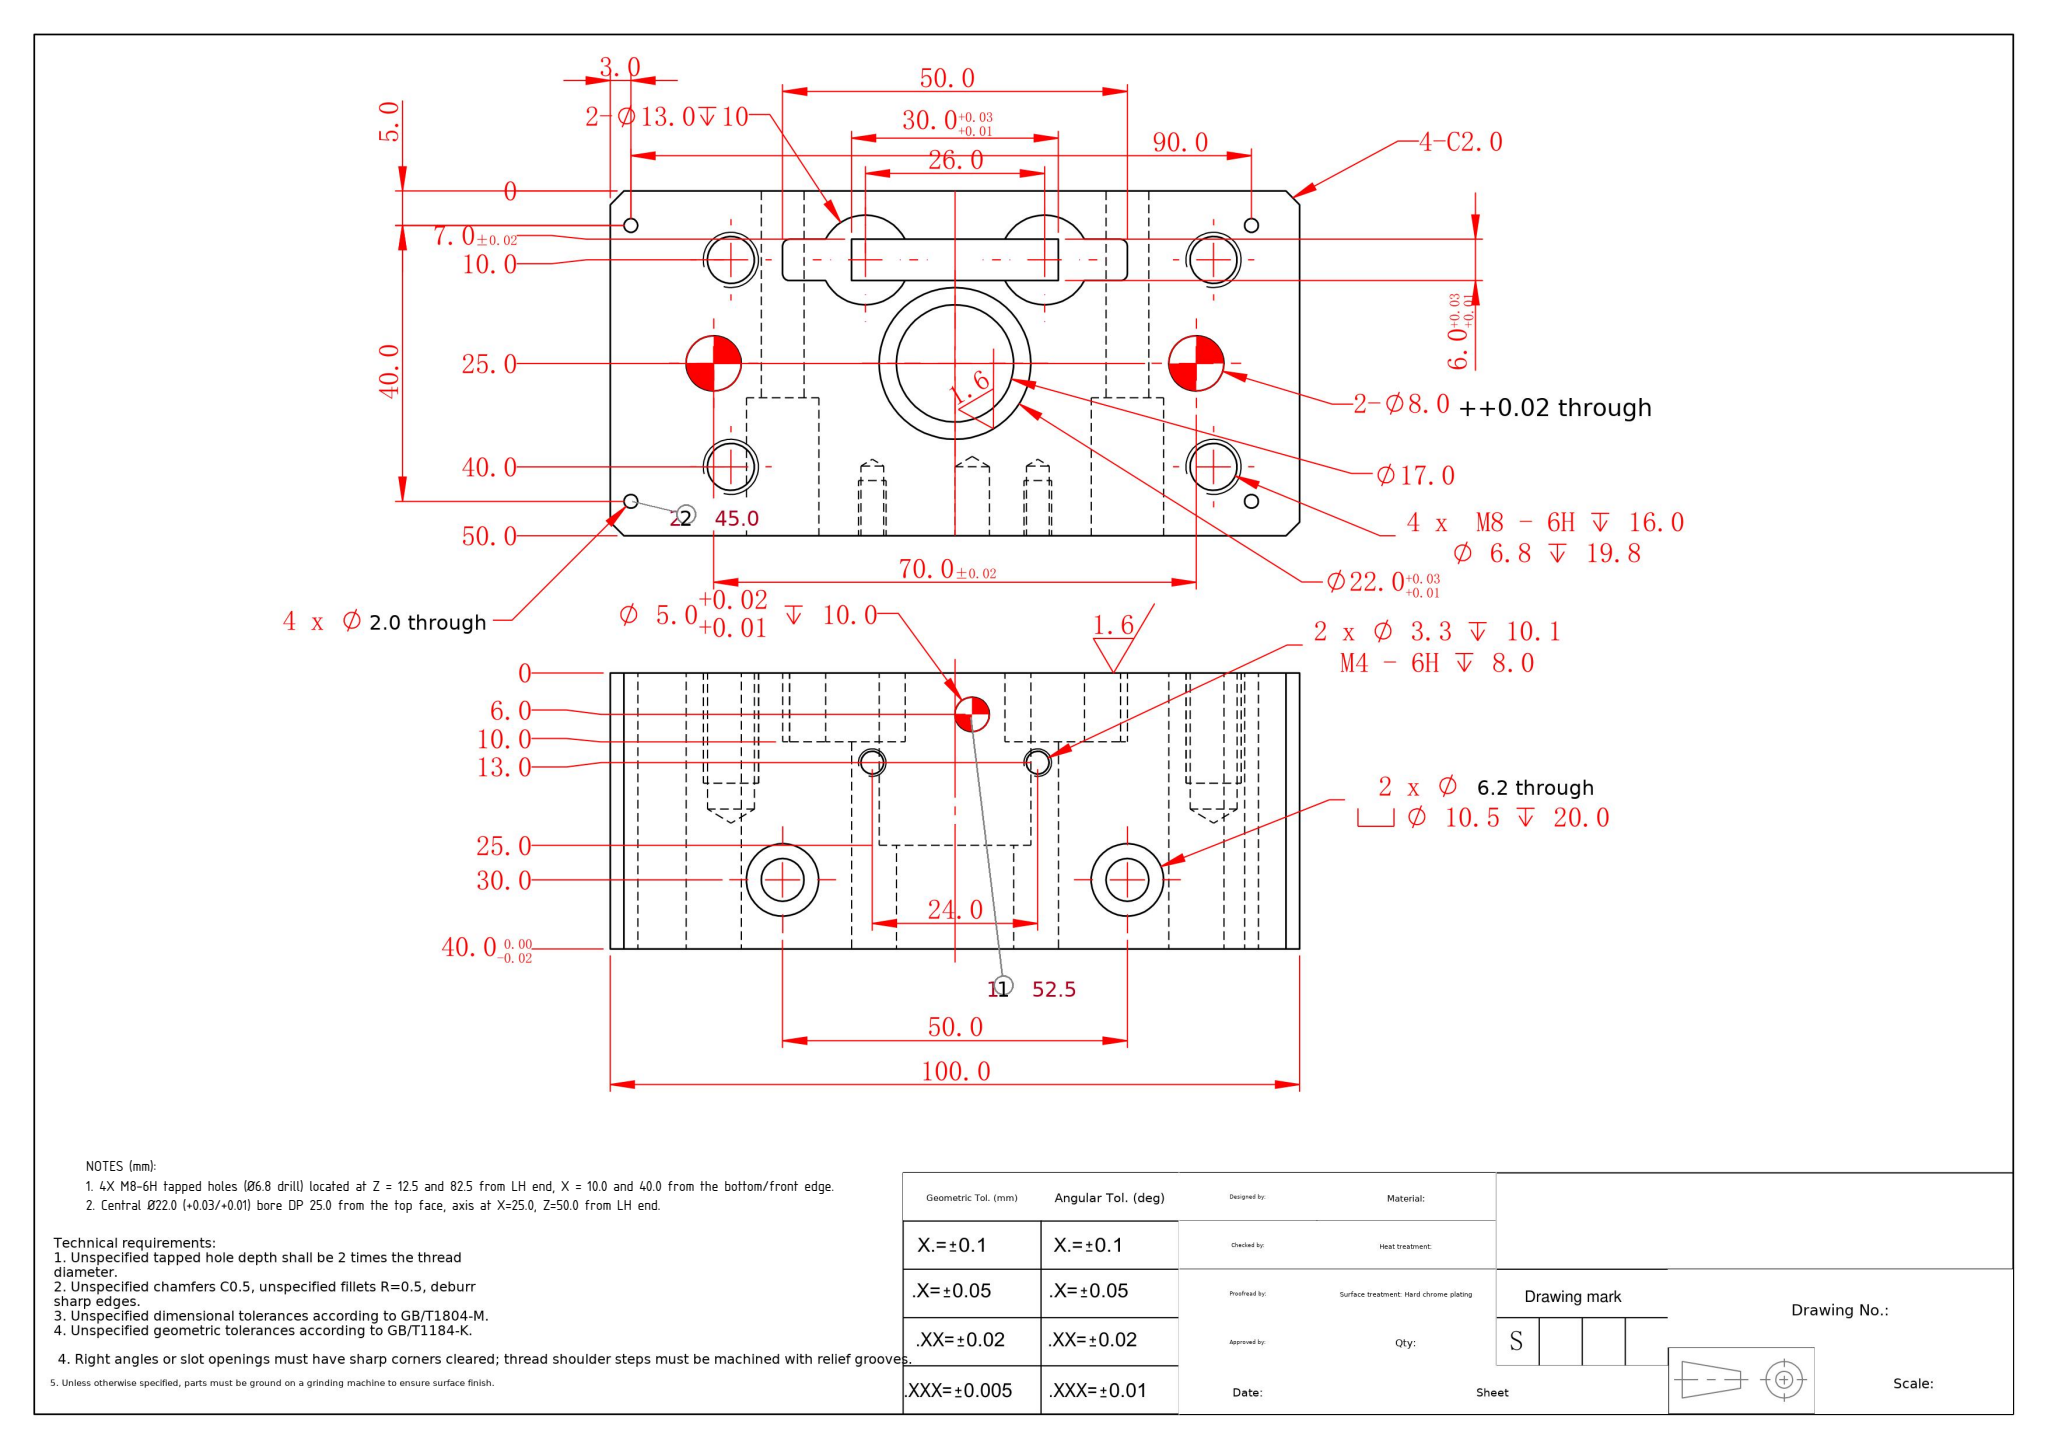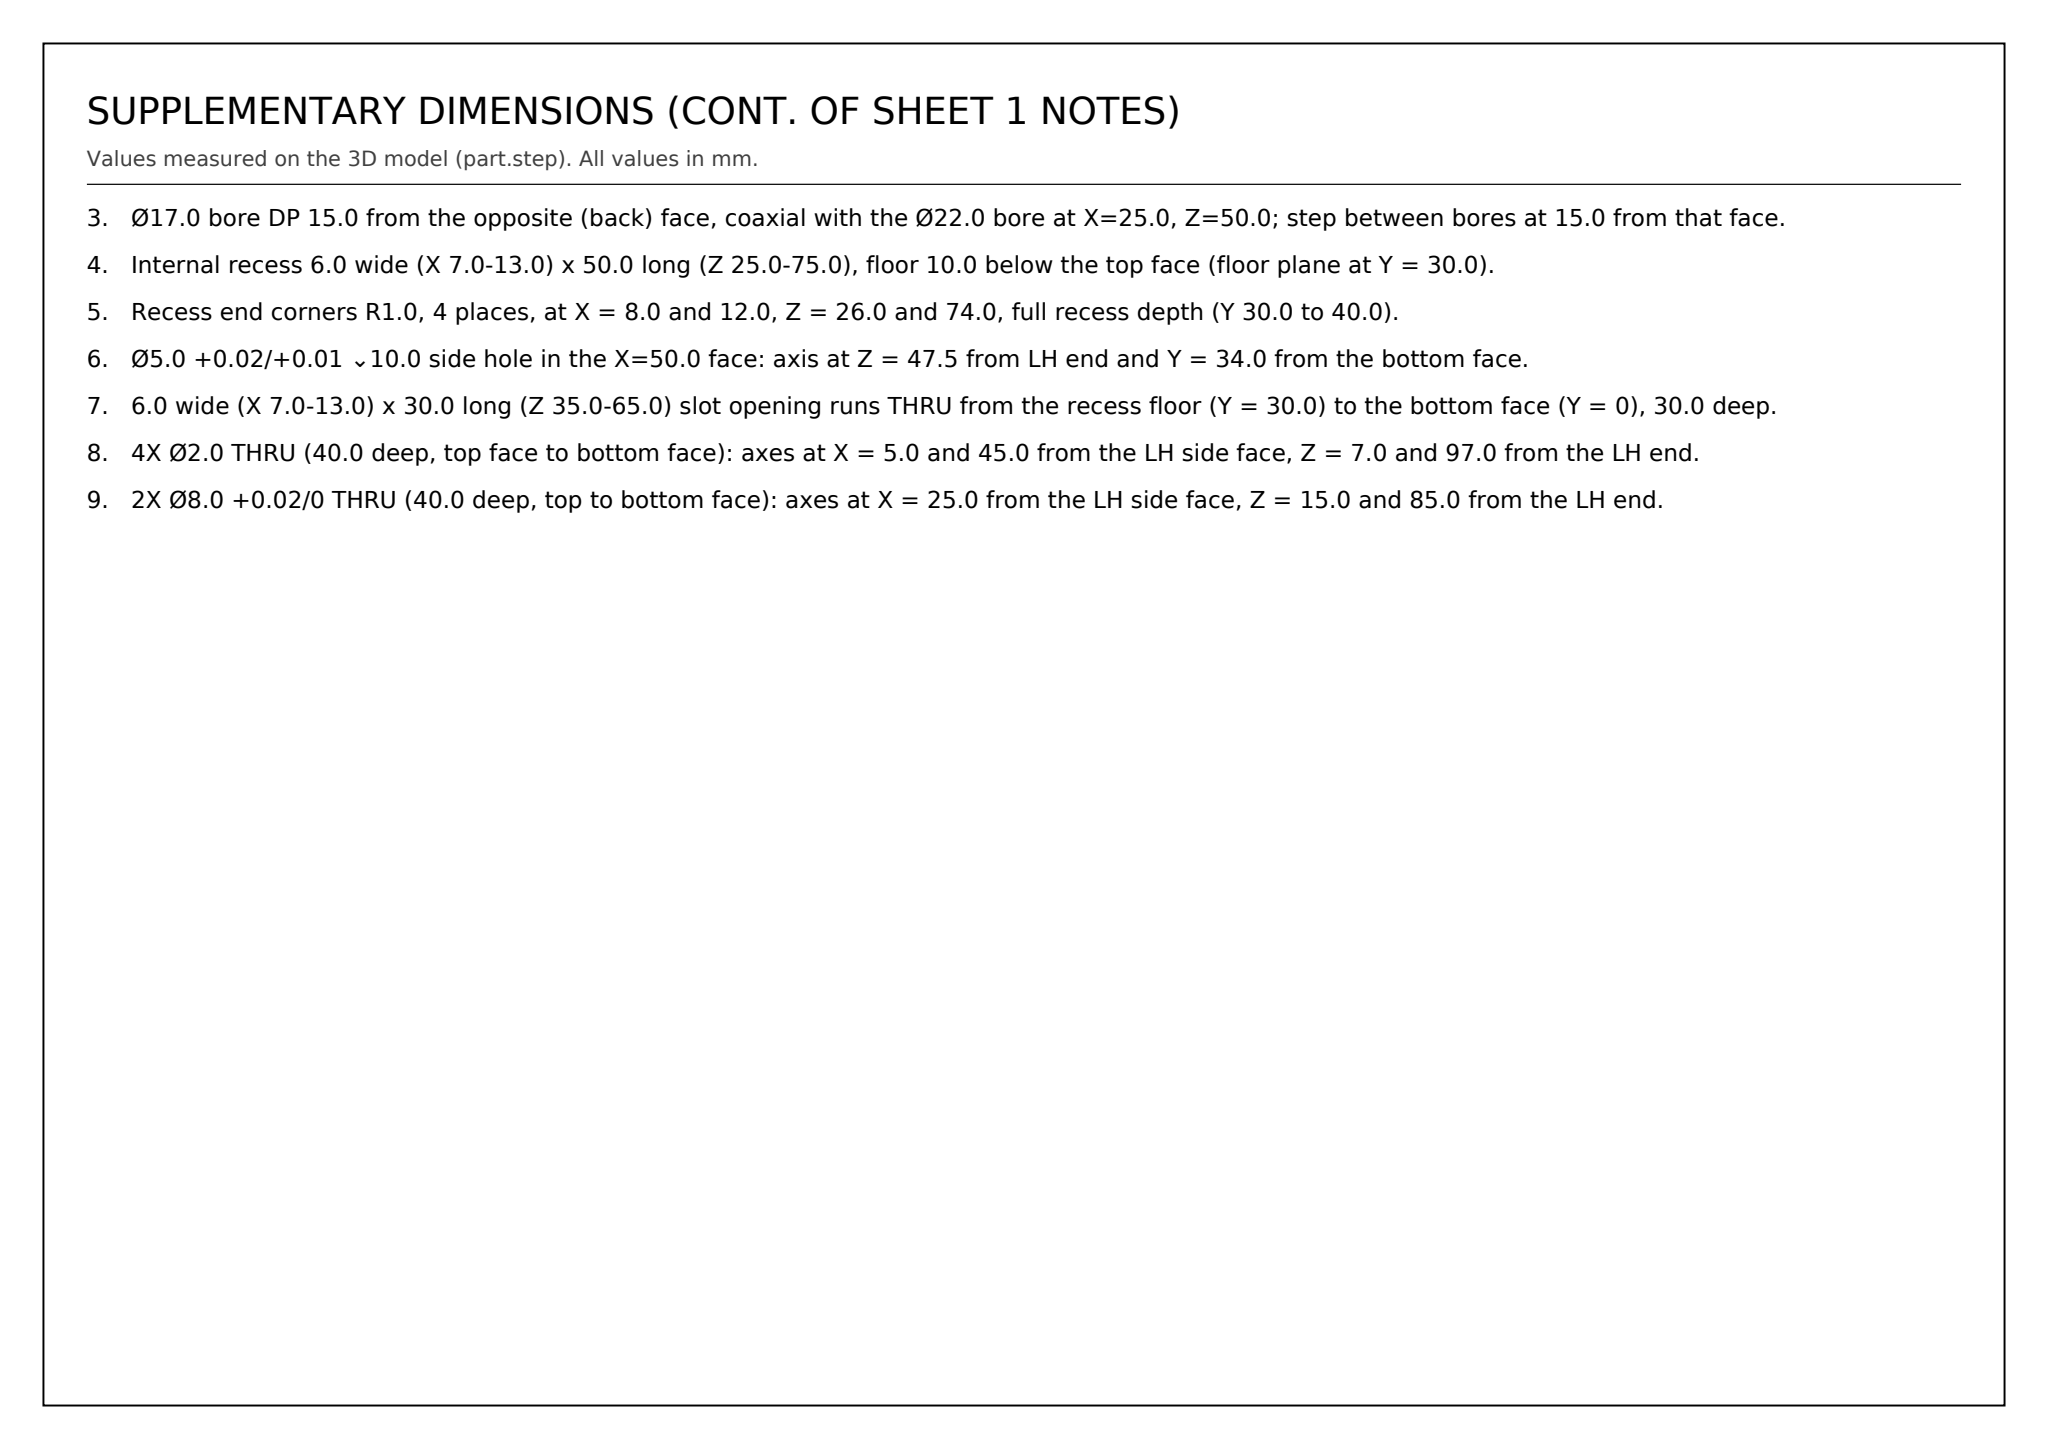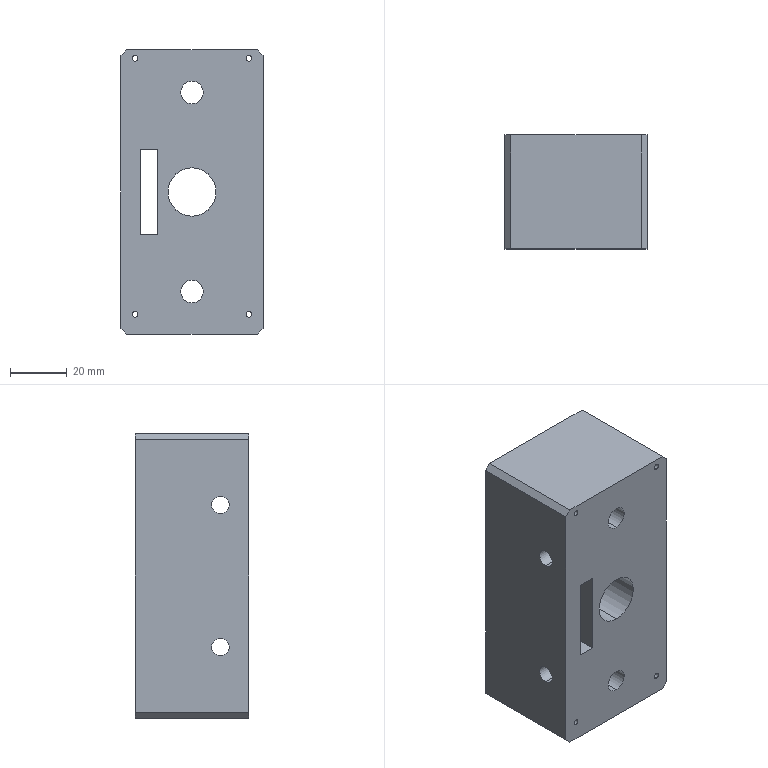Part | SolidWorks | mm | 1 solid | 85 faces | box 50 x 40 x 100 mm | volume 164077 mm3 | cylinder 46 | plane 25 | cone 14 | commonest cylinder face diameters 2 x12 6.8 x8 3.3 x4 10.5 x4 6.2 x4 8 x4 13 x4 5 x2
Drawing notes:
4X M8-6H tapped holes (Ø6.8 drill) located at Z = 12.5 and 82.5 from LH end, X = 10.0 and 40.0 from the bottom/front edge. | from the solid: cylinders: hole/bore dia 6.8, axis y, positions [10.0,null,12.5], [10.0,null,82.5], [40.0,null,12.5], [40.0,null,82.5]
Central Ø22.0 (+0.03/+0.01) bore DP 25.0 from the top face, axis at X=25.0, Z=50.0 from LH end. | from the solid: cylinders: hole/bore dia 22.0, axis y at [25.0,null,50.0], from 15.0 to 40.0 (40.0 = top face)
Ø17.0 bore DP 15.0 from the opposite (back) face, coaxial with the Ø22.0 bore at X=25.0, Z=50.0; step between bores at 15.0 from that face. | from the solid: cylinders: hole/bore dia 17.0, axis y at [25.0,null,50.0], from 0.0 to 15.0; axis_plane y=15.0 extent x[14,36] z[39,61]
Internal recess 6.0 wide (X 7.0-13.0) x 50.0 long (Z 25.0-75.0), floor 10.0 below the top face (floor plane at Y = 30.0). | from the solid: axis_planes: y=30.0 floor patches x[3.5,16.5] z[25,42.8] and z[57.2,75]; x=7.0 and x=13.0 walls y[30,40]; z=25.0 and z=75.0 end walls x[8,12] y[30,40]
Recess end corners R1.0, 4 places, at X = 8.0 and 12.0, Z = 26.0 and 74.0, full recess depth (Y 30.0 to 40.0). | from the solid: cylinders: 4x concave arc dia 2.0 (R1.0), axis y, at (x,z) = (8,26),(8,74),(12,26),(12,74), from y=30.0 to y=40.0, arc 90 deg
Ø5.0 +0.02/+0.01 ⌄10.0 side hole in the X=50.0 face: axis at Z = 47.5 from LH end and Y = 34.0 from the bottom face. | from the solid: cylinders: hole/bore dia 5.0, axis x, axis_pos [y 34.0, z 47.5], from 40.0 to 50.0
6.0 wide (X 7.0-13.0) x 30.0 long (Z 35.0-65.0) slot opening runs THRU from the recess floor (Y = 30.0) to the bottom face (Y = 0), 30.0 deep. | from the solid: axis_planes x=7.0 and x=13.0 extent y [0.0,40.0] z [35.0,65.0]; z=35.0 and z=65.0 planes extent x [7.0,13.0] y [0.0,30.0]
4X Ø2.0 THRU (40.0 deep, top face to bottom face): axes at X = 5.0 and 45.0 from the LH side face, Z = 7.0 and 97.0 from the LH end. | from the solid: cylinders: four hole/bore dia 2.0, axis y, axis_pos x 5.0/45.0, z 7.0/97.0, from 0.0 to 40.0
2X Ø8.0 +0.02/0 THRU (40.0 deep, top to bottom face): axes at X = 25.0 from the LH side face, Z = 15.0 and 85.0 from the LH end. | from the solid: cylinders: hole/bore dia 8.0, axis y, axis_pos x 25.0, z 15.0 and 85.0, from 0.0 to 40.0